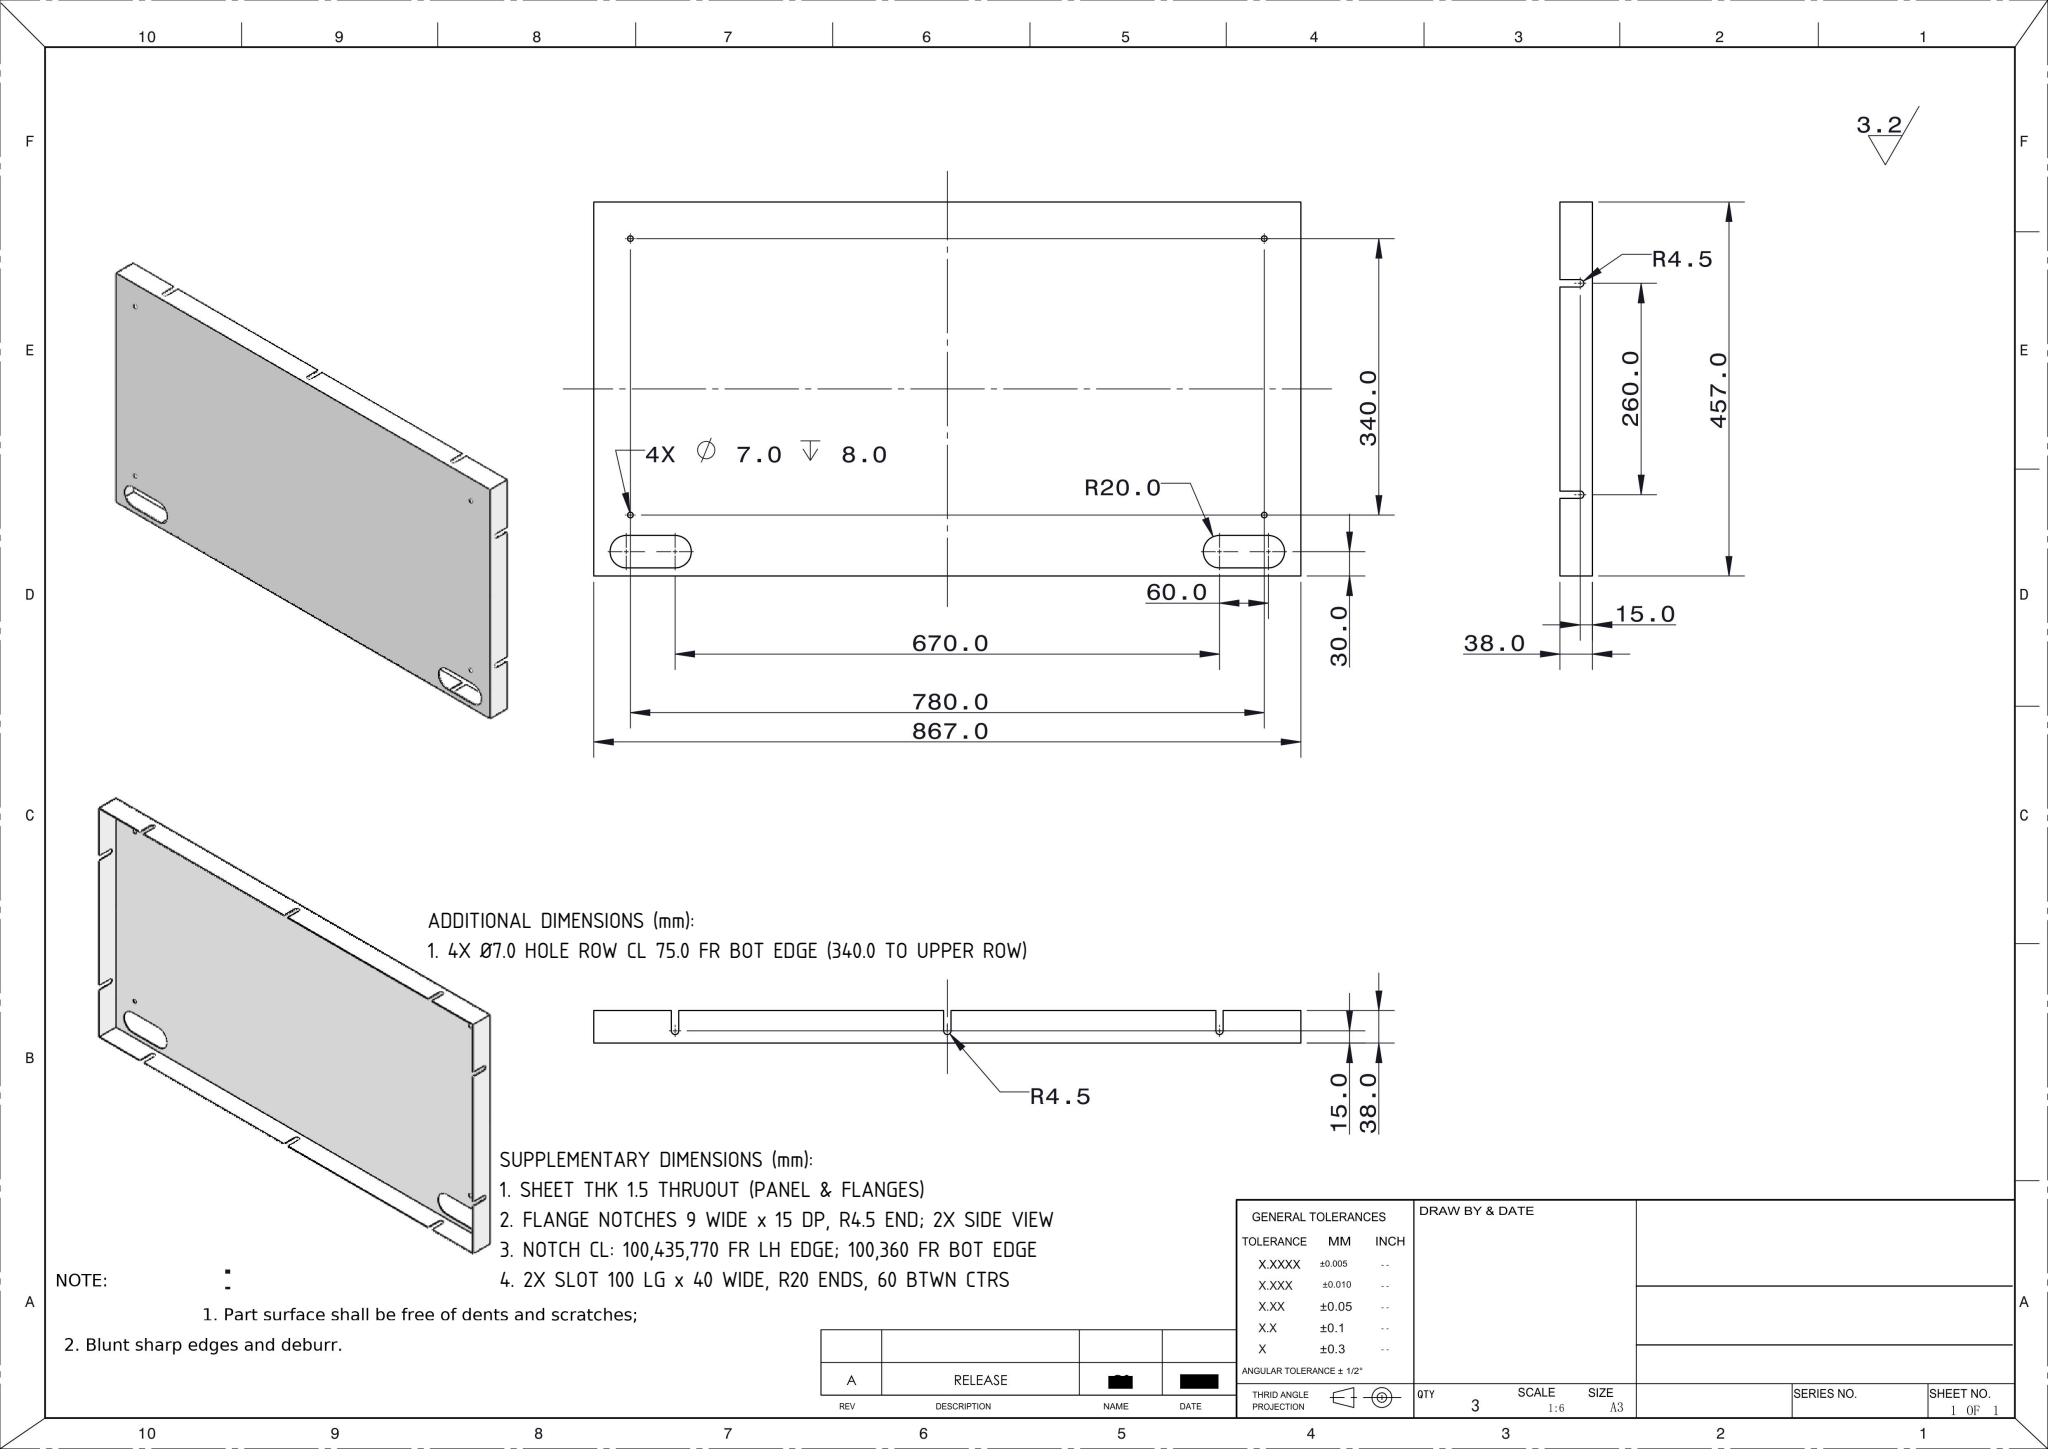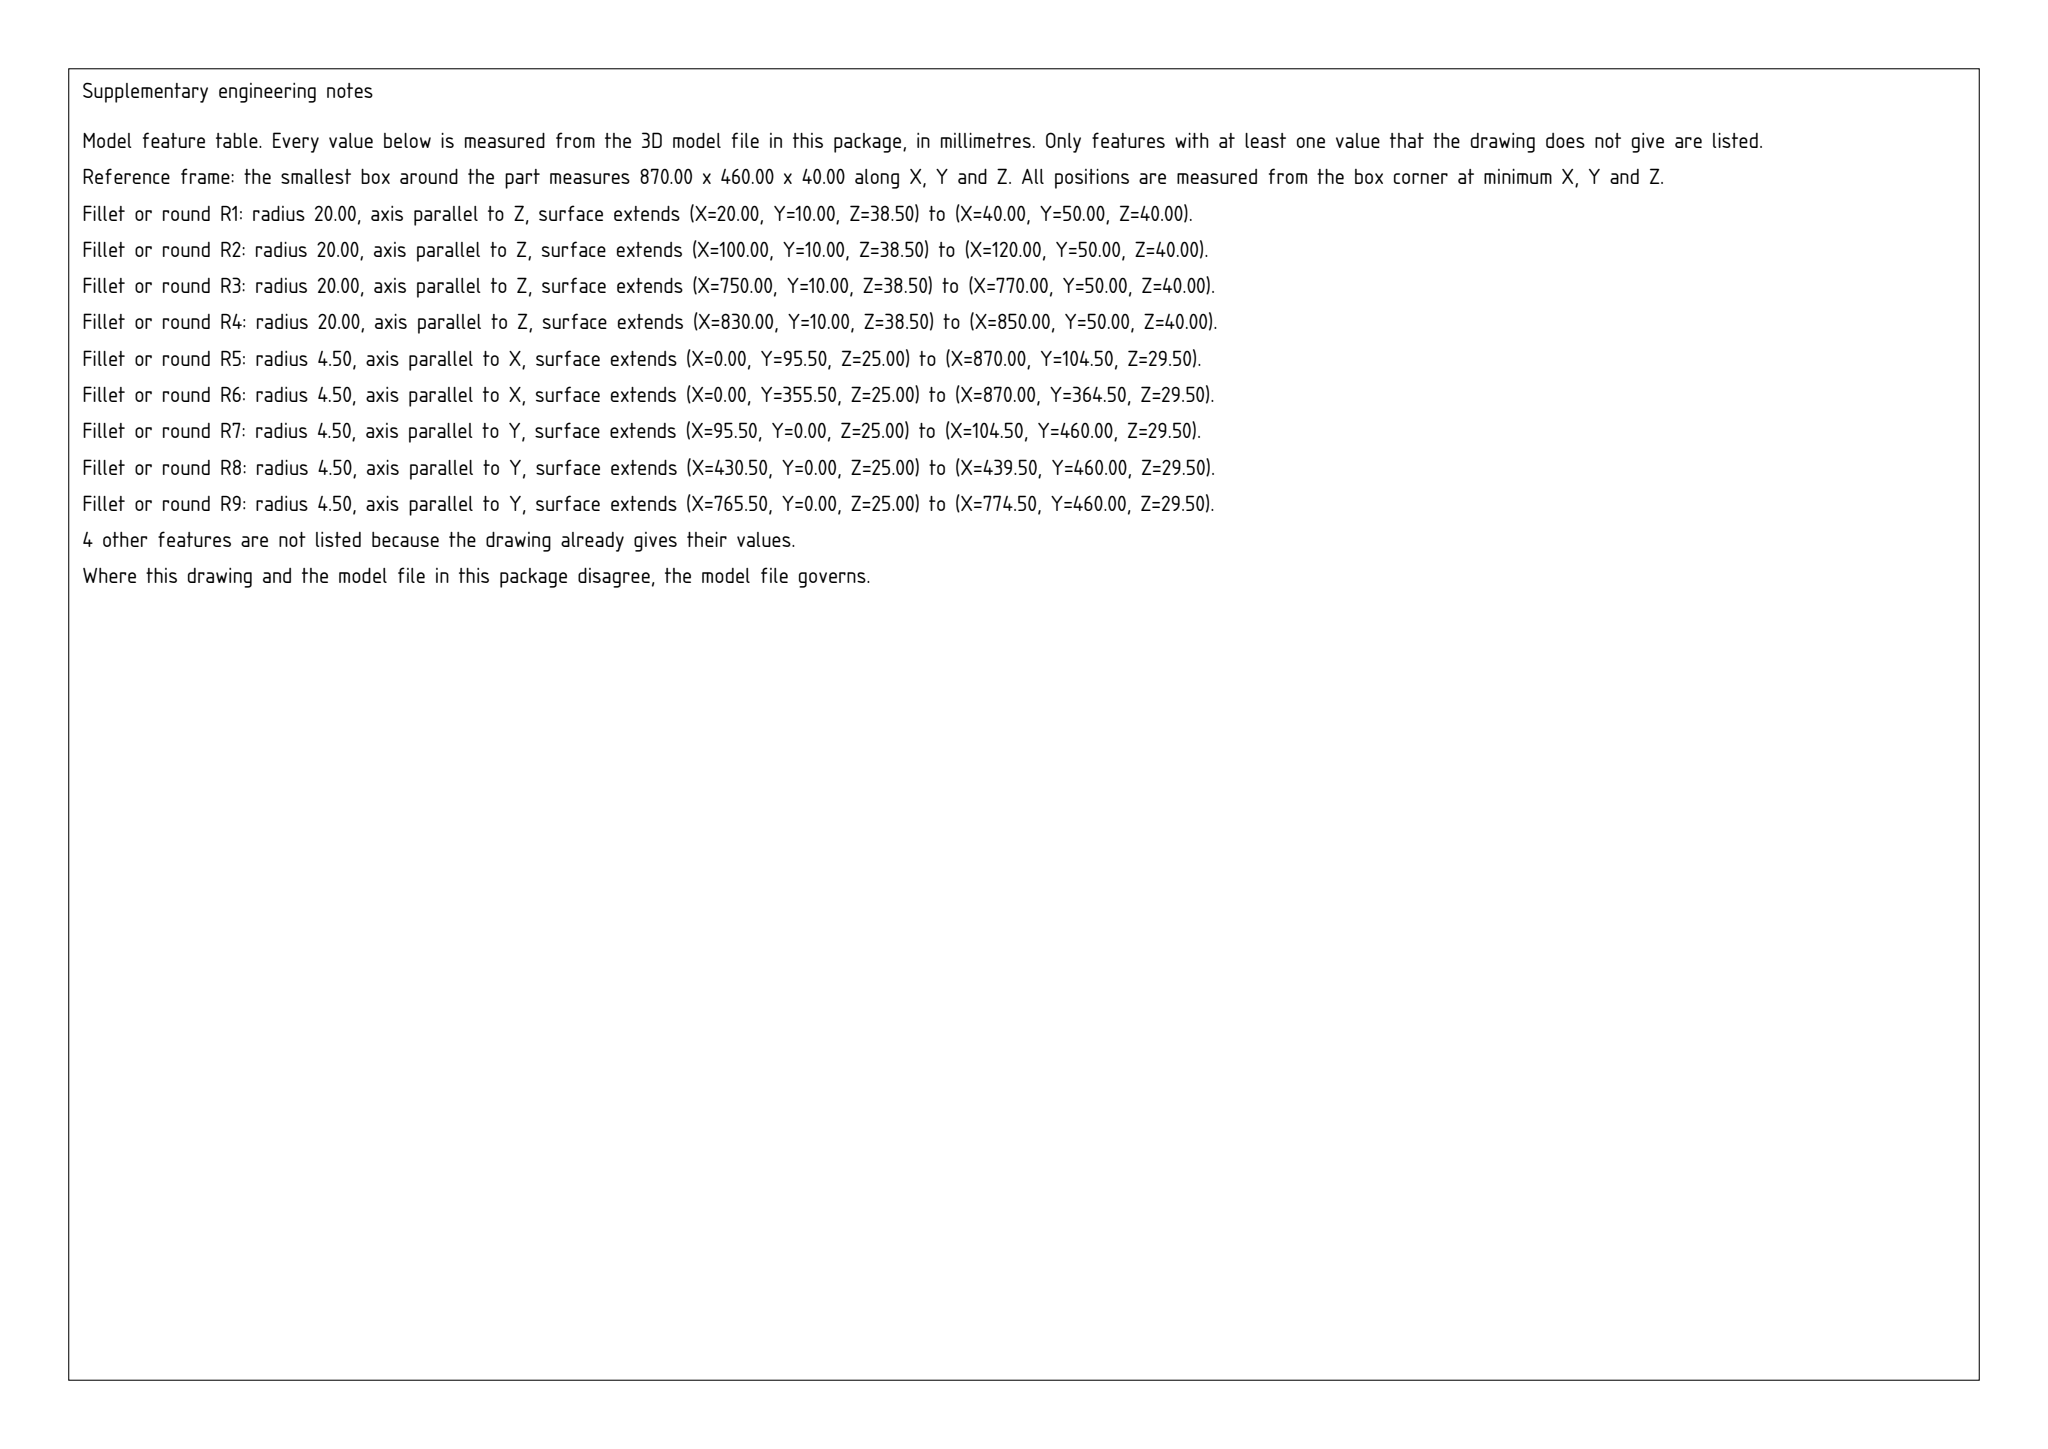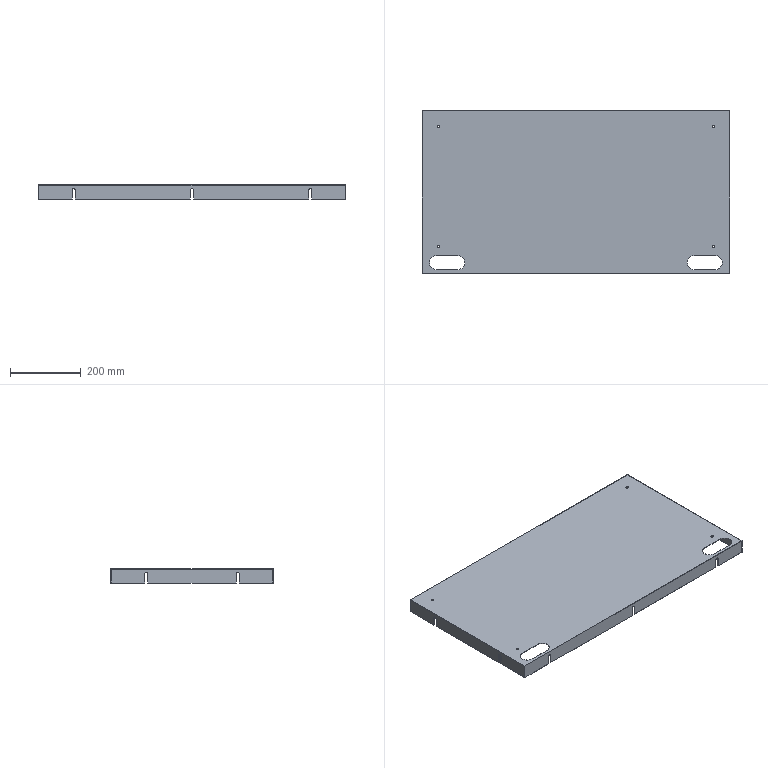Part | SolidWorks | mm | 1 solid | 72 faces | box 870 x 460 x 40 mm | volume 738516 mm3 | plane 44 | cylinder 28 | commonest cylinder face diameters 9 x14 7 x8 40 x6
build123d program:
from build123d import *

# Parameters (mm, degrees)
SKETCH1_W                    = 870
SKETCH1_H                    = 460
BOSS_EXTRUDE1_DEPTH          = 40
SHELL1_T                     = -1.5
CUT_EXTRUDE2_REACH           = 60040.388
F_7_0_7_DIAMETER_HOLE1_D     = 7
F_7_0_7_DIAMETER_HOLE1_DEPTH = 8
F_7_0_7_DIAMETER_HOLE1_TIP   = 2.103
CUT_EXTRUDE4_DEPTH           = 2068.092
CUT_EXTRUDE5_DEPTH           = 60011.876


with BuildPart() as part:
    # Sketch1 → Boss-Extrude1 (new body)
    with BuildSketch(Plane.XY):
        with Locations((-59574.1, 1644.665)):
            Rectangle(SKETCH1_W, SKETCH1_H)
    extrude(amount=BOSS_EXTRUDE1_DEPTH)

    # Shell1
    shell1_openings = [part.faces().sort_by_distance(p)[0] for p in [
        (-59574.1, 1644.665, 0),
    ]]
    offset(amount=SHELL1_T, openings=shell1_openings, kind=Kind.INTERSECTION)

    # Sketch4 → Cut-Extrude2 (cut, up to next)
    with BuildSketch(Plane.XY.offset(40), mode=Mode.PRIVATE) as cut_extrude2_sk1:
        with BuildLine():
            Line((-59239.1, 1424.665), (-59179.1, 1424.665))
            ThreePointArc((-59179.1, 1424.665), (-59159.1, 1444.665), (-59179.1, 1464.665))
            Line((-59179.1, 1464.665), (-59239.1, 1464.665))
            ThreePointArc((-59239.1, 1464.665), (-59259.1, 1444.665), (-59239.1, 1424.665))
        make_face()
    cut_extrude2_tool1 = extrude(cut_extrude2_sk1.sketch, amount=-CUT_EXTRUDE2_REACH, mode=Mode.PRIVATE) & part.part
    # Sketch4 → Cut-Extrude2 (cut, up to next)
    with BuildSketch(Plane.XY.offset(40), mode=Mode.PRIVATE) as cut_extrude2_sk2:
        with BuildLine():
            Line((-59969.1, 1464.665), (-59909.1, 1464.665))
            ThreePointArc((-59909.1, 1464.665), (-59889.1, 1444.665), (-59909.1, 1424.665))
            Line((-59909.1, 1424.665), (-59969.1, 1424.665))
            ThreePointArc((-59969.1, 1424.665), (-59989.1, 1444.665), (-59969.1, 1464.665))
        make_face()
    cut_extrude2_tool2 = extrude(cut_extrude2_sk2.sketch, amount=-CUT_EXTRUDE2_REACH, mode=Mode.PRIVATE) & part.part
    add(cut_extrude2_tool1.solids().sort_by_distance((-59209.1, 1444.665, 40))[0], mode=Mode.SUBTRACT)
    add(cut_extrude2_tool2.solids().sort_by_distance((-59939.1, 1444.665, 40))[0], mode=Mode.SUBTRACT)

    # 7.0 _7_ Diameter Hole1
    with Locations(Plane.XY.offset(40)):
        with Locations((-59964.1, 1489.665), (-59964.1, 1829.665), (-59184.1, 1829.665), (-59184.1, 1489.665)):
            Hole(F_7_0_7_DIAMETER_HOLE1_D / 2, depth=F_7_0_7_DIAMETER_HOLE1_DEPTH)
            with Locations((0, 0, -(F_7_0_7_DIAMETER_HOLE1_DEPTH + F_7_0_7_DIAMETER_HOLE1_TIP / 2))):  # 118° drill point
                Cone(0, F_7_0_7_DIAMETER_HOLE1_D / 2, F_7_0_7_DIAMETER_HOLE1_TIP, mode=Mode.SUBTRACT)

    # Sketch8 → Cut-Extrude4 (cut, through all)
    with BuildSketch(Plane.ZY.offset(60009.1)):
        with BuildLine():
            Line((-5, 1779.165), (25, 1779.165))
            ThreePointArc((25, 1779.165), (29.5, 1774.665), (25, 1770.165))
            Line((25, 1770.165), (-5, 1770.165))
            ThreePointArc((-5, 1770.165), (-9.5, 1774.665), (-5, 1779.165))
        make_face()
        with BuildLine():
            Line((-5, 1510.165), (25, 1510.165))
            ThreePointArc((25, 1510.165), (29.5, 1514.665), (25, 1519.165))
            Line((25, 1519.165), (-5, 1519.165))
            ThreePointArc((-5, 1519.165), (-9.5, 1514.665), (-5, 1510.165))
        make_face()
    extrude(amount=-CUT_EXTRUDE4_DEPTH, mode=Mode.SUBTRACT)

    # Sketch9 → Cut-Extrude5 (cut, through all)
    with BuildSketch(Plane.XZ.offset(-1414.665)):
        with BuildLine():
            Line((-59904.6, 25), (-59904.6, -5))
            ThreePointArc((-59904.6, -5), (-59909.1, -9.5), (-59913.6, -5))
            Line((-59913.6, -5), (-59913.6, 25))
            ThreePointArc((-59913.6, 25), (-59909.1, 29.5), (-59904.6, 25))
        make_face()
        with BuildLine():
            Line((-59234.6, 25), (-59234.6, -5))
            ThreePointArc((-59234.6, -5), (-59239.1, -9.5), (-59243.6, -5))
            Line((-59243.6, -5), (-59243.6, 25))
            ThreePointArc((-59243.6, 25), (-59239.1, 29.5), (-59234.6, 25))
        make_face()
        with BuildLine():
            Line((-59569.6, 25), (-59569.6, -5))
            ThreePointArc((-59569.6, -5), (-59574.1, -9.5), (-59578.6, -5))
            Line((-59578.6, -5), (-59578.6, 25))
            ThreePointArc((-59578.6, 25), (-59574.1, 29.5), (-59569.6, 25))
        make_face()
    extrude(amount=-CUT_EXTRUDE5_DEPTH, mode=Mode.SUBTRACT)


solid = part.part